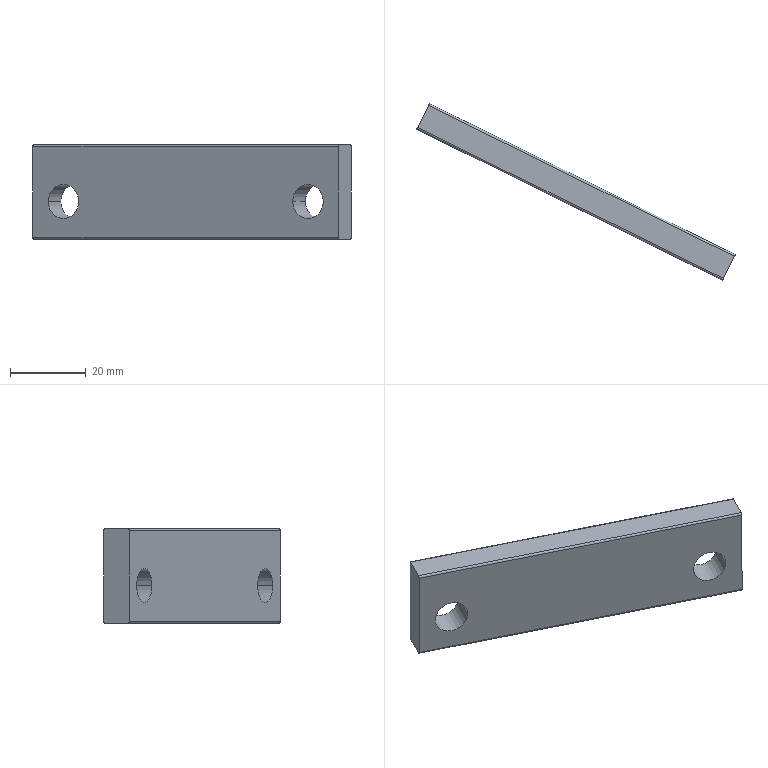Component | SolidWorks | 12AFeedInletSpacer-1 | 1 solid | 14 faces | box 84.01 x 46.6 x 25 mm | volume 15901 mm3 | cylinder 8 | plane 6 | commonest cylinder face diameters 9 x4 1 x4 | material Cr12MoV
build123d program:
from build123d import *

# Parameters (mm, degrees)
SKETCH1_W                    = 90
SKETCH1_H                    = 25
BOSS_EXTRUDE1_DEPTH          = 7.5
F_9_0_9_DIAMETER_HOLE1_D     = 9
F_9_0_9_DIAMETER_HOLE1_DEPTH = 27
F_9_0_9_DIAMETER_HOLE1_TIP   = 2.704
FILLET1_R                    = 0.5


with BuildPart() as part:
    # Sketch1 → Boss-Extrude1 (new body)
    with BuildSketch(Plane.XY):
        Rectangle(SKETCH1_W, SKETCH1_H)
    extrude(amount=BOSS_EXTRUDE1_DEPTH)

    # 9.0 _9_ Diameter Hole1
    with Locations(Plane.XY.offset(7.5)):
        with Locations((-36, 2.5), (36, 2.5)):
            Hole(F_9_0_9_DIAMETER_HOLE1_D / 2, depth=F_9_0_9_DIAMETER_HOLE1_DEPTH)
            with Locations((0, 0, -(F_9_0_9_DIAMETER_HOLE1_DEPTH + F_9_0_9_DIAMETER_HOLE1_TIP / 2))):  # 118° drill point
                Cone(0, F_9_0_9_DIAMETER_HOLE1_D / 2, F_9_0_9_DIAMETER_HOLE1_TIP, mode=Mode.SUBTRACT)

    # Fillet1
    fillet1_edges = [part.edges().sort_by_distance(p)[0] for p in [
        (0, -12.5, 7.5),
        (0, -12.5, 0),
        (0, 12.5, 0),
        (0, 12.5, 7.5),
    ]]
    fillet(fillet1_edges, radius=FILLET1_R)


solid = part.part

# Placed as in the assembly
solid = solid.moved(Location((160.557, 108.624, 630), (90, -26.297, 180)))
STEP:
#1=CARTESIAN_POINT('',(7.751,3.57,24.705));
#2=VERTEX_POINT('',#1);
#3=CARTESIAN_POINT('',(7.433,3.727,24.705));
#4=VERTEX_POINT('',#3);
#5=CARTESIAN_POINT('',(7.592,3.649,24.705));
#6=DIRECTION('',(-0.443,-0.8965,-0.));
#7=DIRECTION('',(-0.8965,0.443,0.));
#8=AXIS2_PLACEMENT_3D('',#5,#6,#7);
#9=CIRCLE('',#8,0.1772);
#10=EDGE_CURVE('',#2,#4,#9,.T.);
#11=ORIENTED_EDGE('',*,*,#10,.F.);
#12=CARTESIAN_POINT('',(7.62,3.305,24.705));
#13=VERTEX_POINT('',#12);
#14=CARTESIAN_POINT('',(7.62,3.305,24.705));
#15=DIRECTION('',(-0.443,-0.8965,-0.));
#16=VECTOR('',#15,39.37);
#17=LINE('',#14,#16);
#18=EDGE_CURVE('',#2,#13,#17,.T.);
#19=ORIENTED_EDGE('',*,*,#18,.T.);
#20=CARTESIAN_POINT('',(7.302,3.462,24.705));
#21=VERTEX_POINT('',#20);
#22=CARTESIAN_POINT('',(7.461,3.384,24.705));
#23=DIRECTION('',(-0.443,-0.8965,-0.));
#24=DIRECTION('',(-0.8965,0.443,0.));
#25=AXIS2_PLACEMENT_3D('',#22,#23,#24);
#26=CIRCLE('',#25,0.1772);
#27=EDGE_CURVE('',#13,#21,#26,.T.);
#28=ORIENTED_EDGE('',*,*,#27,.T.);
#29=CARTESIAN_POINT('',(7.302,3.462,24.705));
#30=DIRECTION('',(-0.443,-0.8965,-0.));
#31=VECTOR('',#30,39.37);
#32=LINE('',#29,#31);
#33=EDGE_CURVE('',#4,#21,#32,.T.);
#34=ORIENTED_EDGE('',*,*,#33,.F.);
#35=EDGE_LOOP('',(#11,#19,#28,#34));
#36=FACE_OUTER_BOUND('',#35,.T.);
#37=CARTESIAN_POINT('',(7.461,3.384,24.705));
#38=DIRECTION('',(-0.443,-0.8965,-0.));
#39=DIRECTION('',(-0.8965,0.443,0.));
#40=AXIS2_PLACEMENT_3D('',#37,#38,#39);
#41=CYLINDRICAL_SURFACE('',#40,0.1772);
#42=ADVANCED_FACE('',(#36),#41,.F.);
#43=CARTESIAN_POINT('',(5.209,4.826,24.705));
#44=VERTEX_POINT('',#43);
#45=CARTESIAN_POINT('',(4.892,4.983,24.705));
#46=VERTEX_POINT('',#45);
#47=CARTESIAN_POINT('',(5.05,4.904,24.705));
#48=DIRECTION('',(-0.443,-0.8965,-0.));
#49=DIRECTION('',(-0.8965,0.443,0.));
#50=AXIS2_PLACEMENT_3D('',#47,#48,#49);
#51=CIRCLE('',#50,0.1772);
#52=EDGE_CURVE('',#44,#46,#51,.T.);
#53=ORIENTED_EDGE('',*,*,#52,.F.);
#54=CARTESIAN_POINT('',(5.079,4.561,24.705));
#55=VERTEX_POINT('',#54);
#56=CARTESIAN_POINT('',(5.079,4.561,24.705));
#57=DIRECTION('',(-0.443,-0.8965,-0.));
#58=VECTOR('',#57,39.37);
#59=LINE('',#56,#58);
#60=EDGE_CURVE('',#44,#55,#59,.T.);
#61=ORIENTED_EDGE('',*,*,#60,.T.);
#62=CARTESIAN_POINT('',(4.761,4.718,24.705));
#63=VERTEX_POINT('',#62);
#64=CARTESIAN_POINT('',(4.92,4.64,24.705));
#65=DIRECTION('',(-0.443,-0.8965,-0.));
#66=DIRECTION('',(-0.8965,0.443,0.));
#67=AXIS2_PLACEMENT_3D('',#64,#65,#66);
#68=CIRCLE('',#67,0.1772);
#69=EDGE_CURVE('',#55,#63,#68,.T.);
#70=ORIENTED_EDGE('',*,*,#69,.T.);
#71=CARTESIAN_POINT('',(4.761,4.718,24.705));
#72=DIRECTION('',(-0.443,-0.8965,-0.));
#73=VECTOR('',#72,39.37);
#74=LINE('',#71,#73);
#75=EDGE_CURVE('',#46,#63,#74,.T.);
#76=ORIENTED_EDGE('',*,*,#75,.F.);
#77=EDGE_LOOP('',(#53,#61,#70,#76));
#78=FACE_OUTER_BOUND('',#77,.T.);
#79=CARTESIAN_POINT('',(4.92,4.64,24.705));
#80=DIRECTION('',(-0.443,-0.8965,-0.));
#81=DIRECTION('',(-0.8965,0.443,0.));
#82=AXIS2_PLACEMENT_3D('',#79,#80,#81);
#83=CYLINDRICAL_SURFACE('',#82,0.1772);
#84=ADVANCED_FACE('',(#78),#83,.F.);
#85=CARTESIAN_POINT('',(4.733,5.061,25.276));
#86=VERTEX_POINT('',#85);
#87=CARTESIAN_POINT('',(4.733,5.061,24.331));
#88=VERTEX_POINT('',#87);
#89=CARTESIAN_POINT('',(4.733,5.061,24.311));
#90=DIRECTION('',(0.,-0.,-1.));
#91=VECTOR('',#90,39.37);
#92=LINE('',#89,#91);
#93=EDGE_CURVE('',#86,#88,#92,.T.);
#94=ORIENTED_EDGE('',*,*,#93,.T.);
#95=CARTESIAN_POINT('',(4.724,5.044,24.311));
#96=VERTEX_POINT('',#95);
#97=CARTESIAN_POINT('',(4.724,5.044,24.331));
#98=DIRECTION('',(-0.8965,0.443,-0.));
#99=DIRECTION('',(-0.443,-0.8965,0.));
#100=AXIS2_PLACEMENT_3D('',#97,#98,#99);
#101=CIRCLE('',#100,0.01969);
#102=EDGE_CURVE('',#88,#96,#101,.T.);
#103=ORIENTED_EDGE('',*,*,#102,.T.);
#104=CARTESIAN_POINT('',(4.611,4.814,24.311));
#105=VERTEX_POINT('',#104);
#106=CARTESIAN_POINT('',(4.602,4.797,24.311));
#107=DIRECTION('',(0.443,0.8965,0.));
#108=VECTOR('',#107,39.37);
#109=LINE('',#106,#108);
#110=EDGE_CURVE('',#105,#96,#109,.T.);
#111=ORIENTED_EDGE('',*,*,#110,.F.);
#112=CARTESIAN_POINT('',(4.602,4.797,24.331));
#113=VERTEX_POINT('',#112);
#114=CARTESIAN_POINT('',(4.611,4.814,24.331));
#115=DIRECTION('',(-0.8965,0.443,-0.));
#116=DIRECTION('',(-0.443,-0.8965,0.));
#117=AXIS2_PLACEMENT_3D('',#114,#115,#116);
#118=CIRCLE('',#117,0.01969);
#119=EDGE_CURVE('',#105,#113,#118,.T.);
#120=ORIENTED_EDGE('',*,*,#119,.T.);
#121=CARTESIAN_POINT('',(4.602,4.797,25.276));
#122=VERTEX_POINT('',#121);
#123=CARTESIAN_POINT('',(4.602,4.797,24.311));
#124=DIRECTION('',(0.,-0.,-1.));
#125=VECTOR('',#124,39.37);
#126=LINE('',#123,#125);
#127=EDGE_CURVE('',#122,#113,#126,.T.);
#128=ORIENTED_EDGE('',*,*,#127,.F.);
#129=CARTESIAN_POINT('',(4.611,4.814,25.295));
#130=VERTEX_POINT('',#129);
#131=CARTESIAN_POINT('',(4.611,4.814,25.276));
#132=DIRECTION('',(-0.8965,0.443,-0.));
#133=DIRECTION('',(-0.443,-0.8965,0.));
#134=AXIS2_PLACEMENT_3D('',#131,#132,#133);
#135=CIRCLE('',#134,0.01969);
#136=EDGE_CURVE('',#122,#130,#135,.T.);
#137=ORIENTED_EDGE('',*,*,#136,.T.);
#138=CARTESIAN_POINT('',(4.724,5.044,25.295));
#139=VERTEX_POINT('',#138);
#140=CARTESIAN_POINT('',(4.602,4.797,25.295));
#141=DIRECTION('',(0.443,0.8965,0.));
#142=VECTOR('',#141,39.37);
#143=LINE('',#140,#142);
#144=EDGE_CURVE('',#130,#139,#143,.T.);
#145=ORIENTED_EDGE('',*,*,#144,.T.);
#146=CARTESIAN_POINT('',(4.724,5.044,25.276));
#147=DIRECTION('',(-0.8965,0.443,-0.));
#148=DIRECTION('',(-0.443,-0.8965,0.));
#149=AXIS2_PLACEMENT_3D('',#146,#147,#148);
#150=CIRCLE('',#149,0.01969);
#151=EDGE_CURVE('',#139,#86,#150,.T.);
#152=ORIENTED_EDGE('',*,*,#151,.T.);
#153=EDGE_LOOP('',(#94,#103,#111,#120,#128,#137,#145,#152));
#154=FACE_OUTER_BOUND('',#153,.T.);
#155=CARTESIAN_POINT('',(4.602,4.797,24.311));
#156=DIRECTION('',(0.8965,-0.443,0.));
#157=DIRECTION('',(-0.443,-0.8965,-0.));
#158=AXIS2_PLACEMENT_3D('',#155,#156,#157);
#159=PLANE('',#158);
#160=ADVANCED_FACE('',(#154),#159,.F.);
#161=ORIENTED_EDGE('',*,*,#110,.T.);
#162=CARTESIAN_POINT('',(7.901,3.474,24.311));
#163=VERTEX_POINT('',#162);
#164=CARTESIAN_POINT('',(7.901,3.474,24.311));
#165=DIRECTION('',(0.8965,-0.443,0.));
#166=VECTOR('',#165,39.37);
#167=LINE('',#164,#166);
#168=EDGE_CURVE('',#96,#163,#167,.T.);
#169=ORIENTED_EDGE('',*,*,#168,.T.);
#170=CARTESIAN_POINT('',(7.787,3.245,24.311));
#171=VERTEX_POINT('',#170);
#172=CARTESIAN_POINT('',(7.779,3.227,24.311));
#173=DIRECTION('',(0.443,0.8965,0.));
#174=VECTOR('',#173,39.37);
#175=LINE('',#172,#174);
#176=EDGE_CURVE('',#171,#163,#175,.T.);
#177=ORIENTED_EDGE('',*,*,#176,.F.);
#178=CARTESIAN_POINT('',(4.611,4.814,24.311));
#179=DIRECTION('',(-0.8965,0.443,-0.));
#180=VECTOR('',#179,39.37);
#181=LINE('',#178,#180);
#182=EDGE_CURVE('',#171,#105,#181,.T.);
#183=ORIENTED_EDGE('',*,*,#182,.T.);
#184=EDGE_LOOP('',(#161,#169,#177,#183));
#185=FACE_OUTER_BOUND('',#184,.T.);
#186=CARTESIAN_POINT('',(7.779,3.227,24.311));
#187=DIRECTION('',(-0.,0.,1.));
#188=DIRECTION('',(0.443,0.8965,0.));
#189=AXIS2_PLACEMENT_3D('',#186,#187,#188);
#190=PLANE('',#189);
#191=ADVANCED_FACE('',(#185),#190,.F.);
#192=ORIENTED_EDGE('',*,*,#176,.T.);
#193=CARTESIAN_POINT('',(7.909,3.492,24.331));
#194=VERTEX_POINT('',#193);
#195=CARTESIAN_POINT('',(7.901,3.474,24.331));
#196=DIRECTION('',(0.8965,-0.443,0.));
#197=DIRECTION('',(0.,0.,-1.));
#198=AXIS2_PLACEMENT_3D('',#195,#196,#197);
#199=CIRCLE('',#198,0.01969);
#200=EDGE_CURVE('',#163,#194,#199,.T.);
#201=ORIENTED_EDGE('',*,*,#200,.T.);
#202=CARTESIAN_POINT('',(7.909,3.492,25.276));
#203=VERTEX_POINT('',#202);
#204=CARTESIAN_POINT('',(7.909,3.492,24.311));
#205=DIRECTION('',(-0.,0.,1.));
#206=VECTOR('',#205,39.37);
#207=LINE('',#204,#206);
#208=EDGE_CURVE('',#194,#203,#207,.T.);
#209=ORIENTED_EDGE('',*,*,#208,.T.);
#210=CARTESIAN_POINT('',(7.901,3.474,25.295));
#211=VERTEX_POINT('',#210);
#212=CARTESIAN_POINT('',(7.901,3.474,25.276));
#213=DIRECTION('',(0.8965,-0.443,0.));
#214=DIRECTION('',(0.,0.,-1.));
#215=AXIS2_PLACEMENT_3D('',#212,#213,#214);
#216=CIRCLE('',#215,0.01969);
#217=EDGE_CURVE('',#203,#211,#216,.T.);
#218=ORIENTED_EDGE('',*,*,#217,.T.);
#219=CARTESIAN_POINT('',(7.787,3.245,25.295));
#220=VERTEX_POINT('',#219);
#221=CARTESIAN_POINT('',(7.779,3.227,25.295));
#222=DIRECTION('',(0.443,0.8965,0.));
#223=VECTOR('',#222,39.37);
#224=LINE('',#221,#223);
#225=EDGE_CURVE('',#220,#211,#224,.T.);
#226=ORIENTED_EDGE('',*,*,#225,.F.);
#227=CARTESIAN_POINT('',(7.779,3.227,25.276));
#228=VERTEX_POINT('',#227);
#229=CARTESIAN_POINT('',(7.787,3.245,25.276));
#230=DIRECTION('',(0.8965,-0.443,0.));
#231=DIRECTION('',(0.,0.,-1.));
#232=AXIS2_PLACEMENT_3D('',#229,#230,#231);
#233=CIRCLE('',#232,0.01969);
#234=EDGE_CURVE('',#220,#228,#233,.T.);
#235=ORIENTED_EDGE('',*,*,#234,.T.);
#236=CARTESIAN_POINT('',(7.779,3.227,24.331));
#237=VERTEX_POINT('',#236);
#238=CARTESIAN_POINT('',(7.779,3.227,24.311));
#239=DIRECTION('',(-0.,0.,1.));
#240=VECTOR('',#239,39.37);
#241=LINE('',#238,#240);
#242=EDGE_CURVE('',#237,#228,#241,.T.);
#243=ORIENTED_EDGE('',*,*,#242,.F.);
#244=CARTESIAN_POINT('',(7.787,3.245,24.331));
#245=DIRECTION('',(0.8965,-0.443,0.));
#246=DIRECTION('',(0.,0.,-1.));
#247=AXIS2_PLACEMENT_3D('',#244,#245,#246);
#248=CIRCLE('',#247,0.01969);
#249=EDGE_CURVE('',#237,#171,#248,.T.);
#250=ORIENTED_EDGE('',*,*,#249,.T.);
#251=EDGE_LOOP('',(#192,#201,#209,#218,#226,#235,#243,#250));
#252=FACE_OUTER_BOUND('',#251,.T.);
#253=CARTESIAN_POINT('',(7.779,3.227,24.311));
#254=DIRECTION('',(-0.8965,0.443,-0.));
#255=DIRECTION('',(0.,-0.,-1.));
#256=AXIS2_PLACEMENT_3D('',#253,#254,#255);
#257=PLANE('',#256);
#258=ADVANCED_FACE('',(#252),#257,.F.);
#259=ORIENTED_EDGE('',*,*,#225,.T.);
#260=CARTESIAN_POINT('',(7.901,3.474,25.295));
#261=DIRECTION('',(-0.8965,0.443,-0.));
#262=VECTOR('',#261,39.37);
#263=LINE('',#260,#262);
#264=EDGE_CURVE('',#211,#139,#263,.T.);
#265=ORIENTED_EDGE('',*,*,#264,.T.);
#266=ORIENTED_EDGE('',*,*,#144,.F.);
#267=CARTESIAN_POINT('',(7.787,3.245,25.295));
#268=DIRECTION('',(0.8965,-0.443,0.));
#269=VECTOR('',#268,39.37);
#270=LINE('',#267,#269);
#271=EDGE_CURVE('',#130,#220,#270,.T.);
#272=ORIENTED_EDGE('',*,*,#271,.T.);
#273=EDGE_LOOP('',(#259,#265,#266,#272));
#274=FACE_OUTER_BOUND('',#273,.T.);
#275=CARTESIAN_POINT('',(7.779,3.227,25.295));
#276=DIRECTION('',(0.,-0.,-1.));
#277=DIRECTION('',(-0.443,-0.8965,-0.));
#278=AXIS2_PLACEMENT_3D('',#275,#276,#277);
#279=PLANE('',#278);
#280=ADVANCED_FACE('',(#274),#279,.F.);
#281=CARTESIAN_POINT('',(7.461,3.384,24.705));
#282=DIRECTION('',(-0.443,-0.8965,-0.));
#283=DIRECTION('',(-0.8965,0.443,0.));
#284=AXIS2_PLACEMENT_3D('',#281,#282,#283);
#285=CIRCLE('',#284,0.1772);
#286=EDGE_CURVE('',#21,#13,#285,.T.);
#287=ORIENTED_EDGE('',*,*,#286,.F.);
#288=ORIENTED_EDGE('',*,*,#27,.F.);
#289=EDGE_LOOP('',(#287,#288));
#290=FACE_BOUND('',#289,.T.);
#291=CARTESIAN_POINT('',(4.92,4.64,24.705));
#292=DIRECTION('',(-0.443,-0.8965,-0.));
#293=DIRECTION('',(-0.8965,0.443,0.));
#294=AXIS2_PLACEMENT_3D('',#291,#292,#293);
#295=CIRCLE('',#294,0.1772);
#296=EDGE_CURVE('',#63,#55,#295,.T.);
#297=ORIENTED_EDGE('',*,*,#296,.F.);
#298=ORIENTED_EDGE('',*,*,#69,.F.);
#299=EDGE_LOOP('',(#297,#298));
#300=FACE_BOUND('',#299,.T.);
#301=ORIENTED_EDGE('',*,*,#242,.T.);
#302=CARTESIAN_POINT('',(4.602,4.797,25.276));
#303=DIRECTION('',(-0.8965,0.443,-0.));
#304=VECTOR('',#303,39.37);
#305=LINE('',#302,#304);
#306=EDGE_CURVE('',#228,#122,#305,.T.);
#307=ORIENTED_EDGE('',*,*,#306,.T.);
#308=ORIENTED_EDGE('',*,*,#127,.T.);
#309=CARTESIAN_POINT('',(7.779,3.227,24.331));
#310=DIRECTION('',(0.8965,-0.443,0.));
#311=VECTOR('',#310,39.37);
#312=LINE('',#309,#311);
#313=EDGE_CURVE('',#113,#237,#312,.T.);
#314=ORIENTED_EDGE('',*,*,#313,.T.);
#315=EDGE_LOOP('',(#301,#307,#308,#314));
#316=FACE_OUTER_BOUND('',#315,.T.);
#317=CARTESIAN_POINT('',(6.19,4.012,24.803));
#318=DIRECTION('',(-0.443,-0.8965,-0.));
#319=DIRECTION('',(-0.8965,0.443,-0.));
#320=AXIS2_PLACEMENT_3D('',#317,#318,#319);
#321=PLANE('',#320);
#322=ADVANCED_FACE('',(#290,#300,#316),#321,.T.);
#323=CARTESIAN_POINT('',(7.592,3.649,24.705));
#324=DIRECTION('',(-0.443,-0.8965,-0.));
#325=DIRECTION('',(-0.8965,0.443,0.));
#326=AXIS2_PLACEMENT_3D('',#323,#324,#325);
#327=CIRCLE('',#326,0.1772);
#328=EDGE_CURVE('',#4,#2,#327,.T.);
#329=ORIENTED_EDGE('',*,*,#328,.T.);
#330=ORIENTED_EDGE('',*,*,#10,.T.);
#331=EDGE_LOOP('',(#329,#330));
#332=FACE_BOUND('',#331,.T.);
#333=CARTESIAN_POINT('',(5.05,4.904,24.705));
#334=DIRECTION('',(-0.443,-0.8965,-0.));
#335=DIRECTION('',(-0.8965,0.443,0.));
#336=AXIS2_PLACEMENT_3D('',#333,#334,#335);
#337=CIRCLE('',#336,0.1772);
#338=EDGE_CURVE('',#46,#44,#337,.T.);
#339=ORIENTED_EDGE('',*,*,#338,.T.);
#340=ORIENTED_EDGE('',*,*,#52,.T.);
#341=EDGE_LOOP('',(#339,#340));
#342=FACE_BOUND('',#341,.T.);
#343=ORIENTED_EDGE('',*,*,#208,.F.);
#344=CARTESIAN_POINT('',(6.321,4.277,24.331));
#345=DIRECTION('',(-0.8965,0.443,-0.));
#346=VECTOR('',#345,39.37);
#347=LINE('',#344,#346);
#348=EDGE_CURVE('',#194,#88,#347,.T.);
#349=ORIENTED_EDGE('',*,*,#348,.T.);
#350=ORIENTED_EDGE('',*,*,#93,.F.);
#351=CARTESIAN_POINT('',(6.321,4.277,25.276));
#352=DIRECTION('',(0.8965,-0.443,0.));
#353=VECTOR('',#352,39.37);
#354=LINE('',#351,#353);
#355=EDGE_CURVE('',#86,#203,#354,.T.);
#356=ORIENTED_EDGE('',*,*,#355,.T.);
#357=EDGE_LOOP('',(#343,#349,#350,#356));
#358=FACE_OUTER_BOUND('',#357,.T.);
#359=CARTESIAN_POINT('',(6.321,4.277,24.803));
#360=DIRECTION('',(-0.443,-0.8965,-0.));
#361=DIRECTION('',(-0.8965,0.443,-0.));
#362=AXIS2_PLACEMENT_3D('',#359,#360,#361);
#363=PLANE('',#362);
#364=ADVANCED_FACE('',(#332,#342,#358),#363,.F.);
#365=ORIENTED_EDGE('',*,*,#60,.F.);
#366=ORIENTED_EDGE('',*,*,#338,.F.);
#367=ORIENTED_EDGE('',*,*,#75,.T.);
#368=ORIENTED_EDGE('',*,*,#296,.T.);
#369=EDGE_LOOP('',(#365,#366,#367,#368));
#370=FACE_OUTER_BOUND('',#369,.T.);
#371=CARTESIAN_POINT('',(4.92,4.64,24.705));
#372=DIRECTION('',(-0.443,-0.8965,-0.));
#373=DIRECTION('',(-0.8965,0.443,0.));
#374=AXIS2_PLACEMENT_3D('',#371,#372,#373);
#375=CYLINDRICAL_SURFACE('',#374,0.1772);
#376=ADVANCED_FACE('',(#370),#375,.F.);
#377=ORIENTED_EDGE('',*,*,#18,.F.);
#378=ORIENTED_EDGE('',*,*,#328,.F.);
#379=ORIENTED_EDGE('',*,*,#33,.T.);
#380=ORIENTED_EDGE('',*,*,#286,.T.);
#381=EDGE_LOOP('',(#377,#378,#379,#380));
#382=FACE_OUTER_BOUND('',#381,.T.);
#383=CARTESIAN_POINT('',(7.461,3.384,24.705));
#384=DIRECTION('',(-0.443,-0.8965,-0.));
#385=DIRECTION('',(-0.8965,0.443,0.));
#386=AXIS2_PLACEMENT_3D('',#383,#384,#385);
#387=CYLINDRICAL_SURFACE('',#386,0.1772);
#388=ADVANCED_FACE('',(#382),#387,.F.);
#389=ORIENTED_EDGE('',*,*,#102,.F.);
#390=ORIENTED_EDGE('',*,*,#348,.F.);
#391=ORIENTED_EDGE('',*,*,#200,.F.);
#392=ORIENTED_EDGE('',*,*,#168,.F.);
#393=EDGE_LOOP('',(#389,#390,#391,#392));
#394=FACE_OUTER_BOUND('',#393,.T.);
#395=CARTESIAN_POINT('',(7.901,3.474,24.331));
#396=DIRECTION('',(0.8965,-0.443,0.));
#397=DIRECTION('',(-0.443,-0.8965,0.));
#398=AXIS2_PLACEMENT_3D('',#395,#396,#397);
#399=CYLINDRICAL_SURFACE('',#398,0.01969);
#400=ADVANCED_FACE('',(#394),#399,.T.);
#401=ORIENTED_EDGE('',*,*,#217,.F.);
#402=ORIENTED_EDGE('',*,*,#355,.F.);
#403=ORIENTED_EDGE('',*,*,#151,.F.);
#404=ORIENTED_EDGE('',*,*,#264,.F.);
#405=EDGE_LOOP('',(#401,#402,#403,#404));
#406=FACE_OUTER_BOUND('',#405,.T.);
#407=CARTESIAN_POINT('',(7.901,3.474,25.276));
#408=DIRECTION('',(-0.8965,0.443,-0.));
#409=DIRECTION('',(0.443,0.8965,0.));
#410=AXIS2_PLACEMENT_3D('',#407,#408,#409);
#411=CYLINDRICAL_SURFACE('',#410,0.01969);
#412=ADVANCED_FACE('',(#406),#411,.T.);
#413=ORIENTED_EDGE('',*,*,#234,.F.);
#414=ORIENTED_EDGE('',*,*,#271,.F.);
#415=ORIENTED_EDGE('',*,*,#136,.F.);
#416=ORIENTED_EDGE('',*,*,#306,.F.);
#417=EDGE_LOOP('',(#413,#414,#415,#416));
#418=FACE_OUTER_BOUND('',#417,.T.);
#419=CARTESIAN_POINT('',(6.199,4.029,25.276));
#420=DIRECTION('',(0.8965,-0.443,0.));
#421=DIRECTION('',(-0.443,-0.8965,0.));
#422=AXIS2_PLACEMENT_3D('',#419,#420,#421);
#423=CYLINDRICAL_SURFACE('',#422,0.01969);
#424=ADVANCED_FACE('',(#418),#423,.T.);
#425=ORIENTED_EDGE('',*,*,#119,.F.);
#426=ORIENTED_EDGE('',*,*,#182,.F.);
#427=ORIENTED_EDGE('',*,*,#249,.F.);
#428=ORIENTED_EDGE('',*,*,#313,.F.);
#429=EDGE_LOOP('',(#425,#426,#427,#428));
#430=FACE_OUTER_BOUND('',#429,.T.);
#431=CARTESIAN_POINT('',(6.199,4.029,24.331));
#432=DIRECTION('',(-0.8965,0.443,-0.));
#433=DIRECTION('',(0.443,0.8965,0.));
#434=AXIS2_PLACEMENT_3D('',#431,#432,#433);
#435=CYLINDRICAL_SURFACE('',#434,0.01969);
#436=ADVANCED_FACE('',(#430),#435,.T.);
#437=CLOSED_SHELL('',(#42,#84,#160,#191,#258,#280,#322,#364,#376,#388,#400,#412,#424,#436));
#438=MANIFOLD_SOLID_BREP('',#437);
#439=CARTESIAN_POINT('',(0.,0.,0.));
#440=DIRECTION('',(0.,0.,1.));
#441=DIRECTION('',(1.,0.,0.));
#442=AXIS2_PLACEMENT_3D('',#439,#440,#441);
#443=(LENGTH_UNIT()NAMED_UNIT(*)SI_UNIT($,.METRE.));
#444=LENGTH_MEASURE_WITH_UNIT(LENGTH_MEASURE(0.0254),#443);
#445=DIMENSIONAL_EXPONENTS(1.,0.,0.,0.,0.,0.,0.);
#446=(CONVERSION_BASED_UNIT('',#444)LENGTH_UNIT()NAMED_UNIT(#445));
#447=UNCERTAINTY_MEASURE_WITH_UNIT(LENGTH_MEASURE(0.00001),#446,'','');
#448=(NAMED_UNIT(*)PLANE_ANGLE_UNIT()SI_UNIT($,.RADIAN.));
#449=(NAMED_UNIT(*)SI_UNIT($,.STERADIAN.)SOLID_ANGLE_UNIT());
#450=(GEOMETRIC_REPRESENTATION_CONTEXT(3)GLOBAL_UNCERTAINTY_ASSIGNED_CONTEXT((#447))GLOBAL_UNIT_ASSIGNED_CONTEXT((#446,#448,#449))REPRESENTATION_CONTEXT('',''));
#451=ADVANCED_BREP_SHAPE_REPRESENTATION('',(#438,#442),#450);
#452=COLOUR_RGB('',0.7922,0.8196,0.9333);
#453=FILL_AREA_STYLE_COLOUR('',#452);
#454=FILL_AREA_STYLE('',(#453));
#455=SURFACE_STYLE_FILL_AREA(#454);
#456=SURFACE_SIDE_STYLE('',(#455));
#457=SURFACE_STYLE_USAGE(.BOTH.,#456);
#458=PRESENTATION_STYLE_ASSIGNMENT((#457));
#459=STYLED_ITEM('',(#458),#438);
#460=(LENGTH_UNIT()NAMED_UNIT(*)SI_UNIT($,.METRE.));
#461=LENGTH_MEASURE_WITH_UNIT(LENGTH_MEASURE(0.0254),#460);
#462=DIMENSIONAL_EXPONENTS(1.,0.,0.,0.,0.,0.,0.);
#463=(CONVERSION_BASED_UNIT('',#461)LENGTH_UNIT()NAMED_UNIT(#462));
#464=UNCERTAINTY_MEASURE_WITH_UNIT(LENGTH_MEASURE(0.00001),#463,'','');
#465=(NAMED_UNIT(*)PLANE_ANGLE_UNIT()SI_UNIT($,.RADIAN.));
#466=(NAMED_UNIT(*)SI_UNIT($,.STERADIAN.)SOLID_ANGLE_UNIT());
#467=(GEOMETRIC_REPRESENTATION_CONTEXT(3)GLOBAL_UNCERTAINTY_ASSIGNED_CONTEXT((#464))GLOBAL_UNIT_ASSIGNED_CONTEXT((#463,#465,#466))REPRESENTATION_CONTEXT('',''));
#468=MECHANICAL_DESIGN_GEOMETRIC_PRESENTATION_REPRESENTATION('',(#459),#467);
#469=PRESENTATION_LAYER_ASSIGNMENT('','',(#459));